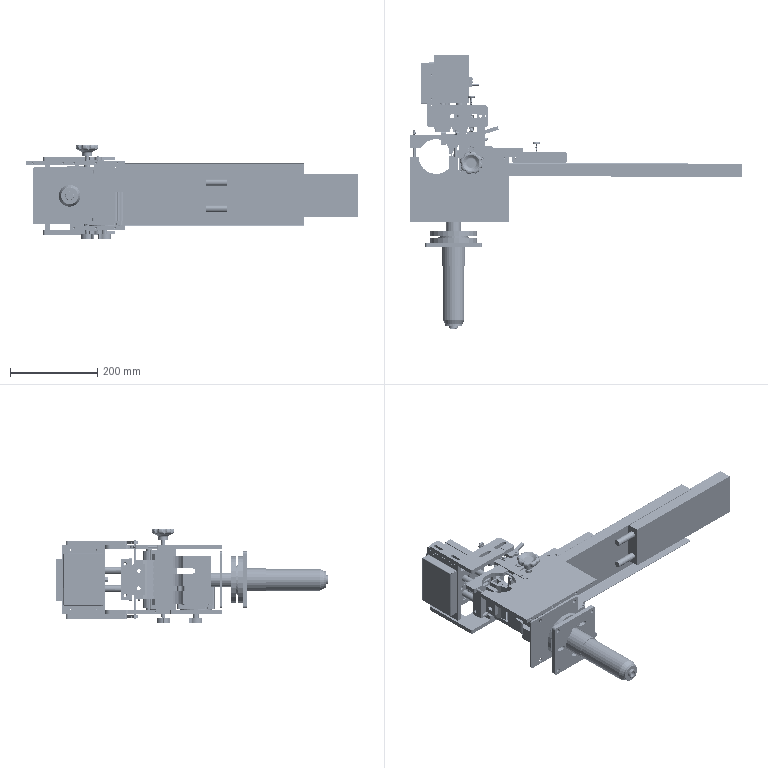Assembly | SolidWorks | mm | 70 component files | 73 solids | 4657 faces | box 762 x 626.5 x 217.5 mm | volume 5183306 mm3 | cylinder 2396 | plane 1290 | sphere 364 | torus 287 | cone 216 | spline 104 | commonest cylinder face diameters 4 x1072 6 x169 9 x90 0.4 x88 10 x69 5 x64 28 x58 30 x56
Bill of materials:
111.1 | 1 |  | Rectangular block-like plate with two holes drilled into one narrow edge face and two small holes through the broad face near one long side.
120.1 | 1 |  | Long slender bar with a thicker block at each end, giving a shallow C/bracket side profile, and four through holes spaced along its length.
121.1 | 1 |  | Thin flat plate whose ends are cut at angles, giving an irregular polygonal outline in one view, with two small through holes near one long edge.
86StepperMotor-XG2.1 | 1 |  | Square-section housing with a wider square flange at the base and a cylindrical shaft sticking out of the flange face; its overall form looks like a motor-style body.
113.1 | 1 |  | Rectangular block with a stepped profile (thick section narrowing through fillets to a thinner section) and two parallel obround through slots.
114.1 | 1 |  | Stepped cylindrical pin with a larger-diameter section, a thin radial collar, and a smaller-diameter section.
115.1 | 1 |  | Flat annular disc/flange with a large central bore and six holes on a circle, alternating between two sizes.
116.1 | 1 |  | Flat annular disc/flange with a large central bore, a step or recess around the bore on one face, and nine holes in three sizes on a circle.
117.1 | 1 |  | Thin flat ring (washer- or shim-like annulus) with a narrow radial width.
118.1 | 1 |  | Plain annular ring, thicker than a thin washer, with a narrow radial wall.
Ultrasonic.1 | 1 |  | Elongated cylindrical body with one end tapering through a conical chamfer to a smaller stepped boss and a small tubular nub with a central bore.
UltrasonicConnectionBlock.1 | 1 |  | Square flat plate with rounded corners, four corner through holes, a large central lobed opening, and three obround slots around the opening.
MainTailstock.1 | 2 |  | Flat, constant-thickness plate with a stepped, offset (Z-like) outline and rounded corners. It has five round through holes in the face and one small hole drilled into a side edge.
Part1.1 | 2 |  | Thick, roughly rectangular block. One end is cut as a concave arc, one corner has a large radius, and there is one round through hole.
ShortBoltM4.1 | 2 |  | Headed threaded fastener shape: a large, thin, disc-shaped head with rounded edges and a smooth (non-knurled) rim, on a coaxial straight shank that has external thread form along most of its length. Looks like a thumb screw or leveling-foot style screw.
ShortBoltM4.1 | 2 |  | Screw-like part: a short, wide disc-shaped head with rounded edges and a long, threaded-looking cylindrical shank. There are plain sections near the head and at the tip.
TailstockAdjustmentPlate.1 | 2 |  | Flat rectangular bar with three equally spaced round through holes in a line. One end is a concave arc and the other end has one large rounded corner.
TailstockAdjustmentSub-Plate.1 | 2 |  | Thick plate with one large rounded corner, a concave arc on the opposite end ending in a small hooked tip, and one round through hole.
TailstockAxisBar.1 | 4 |  | Plain, slender solid cylindrical rod with flat ends.
BladeHolderPlate.1 | 2 |  | Rectangular plate or block with rounded corners and two parallel obround (slotted) through holes.
CoverPlate.1_2 | 1 |  | Thin rectangular plate with rounded corners, four small round holes near the corners, and a large central obround or rounded-rectangle opening.
CoverPlate.1 | 1 |  | Formed thin-wall, sheet-like tray: a shallow rectangular recessed pan with walls, plus outward flanges at two opposite ends. Each flange has two obround slots.
Frame.1 | 2 |  | Flat L-shaped plate with rounded corners and four elongated slots, two along each leg.
FrameCutterBackingPlate.1 | 1 |  | Long, narrow, thin strip with a tab at each end. Each tab has a small round hole and an obround slot. A narrow formed lip or rib runs along one long edge.
FrameFrontMatchingPlate.1 | 1 |  | Plain rectangular bar or block with two round blind holes that appear to have conical drill-point bottoms.
FrameFrontPlate.1 | 1 |  | Thick rectangular plate with a central rectangular through cutout, a pattern of round through holes, and two holes drilled into one narrow edge.
FrameLeftPlate.1 | 1 |  | Flat plate with a stepped outline: a wide rectangular lower section and a narrower arm. It has a long rectangular slot, a large obround cutout, four elongated slots, and several round holes.
FramePlateSlider.1 | 2 |  | Rectangular block with rounded vertical corners, one large round through bore set toward one end, and four corner through holes.
FrameRightPlate.1 | 1 |  | Flat plate with a stepped outline: a wide solid rectangular section and a narrower arm with a long rectangular slot and several round holes. It has the same outline as unnamed part, but without the obround cutout and elongated slots.
GB_T276-94DeepGrooveBallBearing61800.1 | 4 | GCr4 | Ring-shaped assembly of concentric inner and outer rings with a ring of spherical balls between them; it looks like an open ball bearing.
Handle.1 | 2 |  | Straight bar of rectangular section with a semicircular lobe on one side; the lobe holds a round through hole. The lobe blends into the bar with fillets.
HeatingBlock.1 | 1 |  | Plain rectangular block with two parallel cylindrical pins sticking out of one end face.
HeatingBoxCover.1 | 1 |  | Long thin-walled channel (C-shaped section) made of a flat web and two short flanges, with small inner bend radii.
HotKnife.1 | 1 |  | Plate with a row of teeth along one long edge and two round through holes. In profile it tapers toward the toothed edge and has a rectangular notch on the opposite side; it looks like a serrated blade.
HotKnife-Copy.1 | 1 |  | Plate tapering to a single-bevel straight edge, with two round through holes and a rectangular notch in the thicker back portion of the profile; it looks like a straight-edged blade.
KnurledWheel.1 | 1 |  | Round knob with a scalloped (lobed) rim, a shallow dished top, and a conical underside that tapers into a cylindrical hub.
LongBoltM4.1 | 2 |  | Long, slender threaded rod with a flat cylindrical disc head at one end and a short neck between the head and the threads.
PatternedRoller.1 | 1 |  | Cylindrical roller-like body with stepped, smaller-diameter journals extending coaxially from both ends; faint helical lines on the main cylindrical surface.
PipeLockPlate.1 | 1 |  | Flat rectangular plate with a large circular opening at one end, split across the bore; a separate cap block closes the opening and is joined to the plate by two parallel rods with threaded ends, forming a split-bore clamp shape.
PryBarAxis.1 | 1 |  | Long, slender solid cylindrical rod with short modified sections at both ends.
Pulley11.1 | 1 |  | Short cylindrical toothed wheel with evenly spaced rectangular teeth around its outside and a central round through-bore that has one rectangular keyway. Looks like a simplified spur gear, sprocket or timing pulley with straight-sided teeth.
Pulley11.1 | 1 |  | Short cylindrical disk with evenly spaced rectangular teeth around its outside and a central round through-bore.
PunchingKnifeBackingPlate.1 | 2 |  | Flat rectangular plate with rounded corners, an elongated slot near each end, and two small round through-holes between the slots.
RubberRoller.1 | 1 |  | Plain cylindrical body with coaxial stepped journals at both ends.
Spring.1 | 2 |  | Helical coil of round wire with constant coil diameter and uniform pitch, ends left open.
CS1-J().1 | 2 |  | Multi-feature body: a rectangular base block with a raised open-frame upright holding a short cross pin, a long cylindrical rod sticking out sideways, rounded bosses on one face, and a thin hooked lip.
TN32-30 - 30_b.1 | 2 |  | Rectangular block with two parallel stacked bores on one end face, longitudinal grooves on several faces, through-holes on the broad face, and a protruding hex-shaped fitting.
TN32-30_fp.1 | 2 |  | Rectangular end plate carrying two parallel cylindrical rods, each ending in a larger-diameter cylindrical head.
Mates:
1. symmetric | FrameLeftPlate.1-1 face at (2, 116, -70) dir (0, 0, 1) | FrameRightPlate.1-1 face at (2, 116, 70) dir (0, 0, -1) | assembly plane at (0, 0, 0) dir (0, 0, 1)
2. concentric | FrameLeftPlate.1-1 face at (67, 146, -70) dir (0, 0, 1) r 2.75 | 111.1-1 face at (67, 146, -70) dir (0, 0, -1) r 2.1
3. width | 111.1-1 face at (127, 150, -70) dir (0, 0, -1) | 111.1-1 face at (127, 150, 70) dir (0, 0, 1) | FrameLeftPlate.1-1 face at (2, 116, -70) dir (0, 0, 1) | FrameRightPlate.1-1 face at (2, 116, 70) dir (0, 0, -1)
4. concentric | FrameRightPlate.1-1 face at (17, 116.5, 79.4) dir (0, 0, 1) r 2.75 | FrameFrontMatchingPlate.1-1 face at (17, 116.5, 70) dir (0, 0, 1) r 2.1
5. concentric | FrameLeftPlate.1-1 face at (17, 131.5, -70) dir (0, 0, 1) r 2.75 | FrameFrontMatchingPlate.1-1 face at (17, 131.5, -70) dir (0, 0, -1) r 2.1
6. width | FrameFrontMatchingPlate.1-1 face at (21, 146.5, -70) dir (0, 0, -1) | FrameFrontMatchingPlate.1-1 face at (21, 146.5, 70) dir (0, 0, 1) | FrameLeftPlate.1-1 face at (2, 116, -70) dir (0, 0, 1) | FrameRightPlate.1-1 face at (2, 116, 70) dir (0, 0, -1)
7. coincident | FrameLeftPlate.1-1 face at (10, 268, -70) dir (0, 1, 0) | Frame.1-1 face at (69.5, 268, -79.4) dir (0, 1, 0)
8. coincident | FrameLeftPlate.1-1 face at (2, 116, -79.4) dir (0, 0, -1) | Frame.1-1 face at (69.5, 258, -79.4) dir (0, 0, 1)
9. coincident | FrameRightPlate.1-1 face at (10, 268, 79.4) dir (0, 1, 0) | Frame.1-2 face at (69.5, 268, 89.4) dir (0, 1, 0)
10. coincident | FrameRightPlate.1-1 face at (2, 116, 79.4) dir (0, 0, 1) | Frame.1-2 face at (69.5, 258, 79.4) dir (0, 0, -1)
11. width | FrameFrontPlate.1-1 face at (-55.5, 363, -79.4) dir (0, 0, -1) | FrameFrontPlate.1-1 face at (-55.5, 363, 79.4) dir (0, 0, 1) | Frame.1-1 face at (69.5, 258, -79.4) dir (0, 0, 1) | Frame.1-2 face at (69.5, 258, 79.4) dir (0, 0, -1)
12. coincident | FrameFrontMatchingPlate.1-1 face at (21, 146.5, 70) dir (0, 1, 0) | FrameCutterBackingPlate.1-1 face at (0, 146.5, -69) dir (0, -1, 0)
13. width | FrameCutterBackingPlate.1-1 face at (34, 150.5, 69) dir (0, 0, 1) | FrameCutterBackingPlate.1-1 face at (34, 150.5, -69) dir (0, 0, -1) | FrameRightPlate.1-1 face at (2, 116, 70) dir (0, 0, -1) | FrameLeftPlate.1-1 face at (2, 116, -70) dir (0, 0, 1)
14. coincident | 120.1-1 face at (2, 150.5, 69) dir (0, -1, 0) | FrameCutterBackingPlate.1-1 face at (0, 150.5, -69) dir (0, 1, 0)
15. concentric | 120.1-1 face at (8, 150.5, -63) dir (0, -1, 0) r 2.5 | FrameCutterBackingPlate.1-1 face at (8, 146.5, -63) dir (0, -1, 0) r 1.65
16. coincident | 120.1-1 face at (0, 159.5, 59) dir (0, -1, 0) | 121.1-1 face at (5, 159.5, -58) dir (0, 1, 0)
17. concentric | FrameRightPlate.1-1 face at (40.5, 135, 79.4) dir (0, 0, -1) r 9.5 | PatternedRoller.1-1 face at (40.5, 135, 70) dir (0, 0, -1) r 7
18. width | PatternedRoller.1-1 face at (40.5, 135, -65) dir (0, 0, -1) | PatternedRoller.1-1 face at (40.5, 135, 65) dir (0, 0, 1) | FrameRightPlate.1-1 face at (2, 116, 79.4) dir (0, 0, 1) | FrameLeftPlate.1-1 face at (2, 116, -79.4) dir (0, 0, -1)
19. concentric | FrameRightPlate.1-1 face at (40.5, 268, 74.7) dir (0, 1, 0) r 2.1 | LongBoltM4.1-1 face at (40.5, 290, 74.7) dir (0, -1, 0) r 8
20. distance | FrameRightPlate.1-1 face at (10, 268, 79.4) dir (0, 1, 0) | LongBoltM4.1-1 face at (40.5, 290, 74.7) dir (0, 1, 0)
21. coincident | Spring.1-1 plane at (40.5, 207.5, 74.7) dir (0.3882, 0, 0.9216) | LongBoltM4.1-1 plane at (40.5, 205, 74.7) dir (0.3882, 0, 0.9216)
22. coincident | Spring.1-1 plane at (40.5, 207.5, 74.7) dir (0.9216, 0, -0.3882) | LongBoltM4.1-1 plane at (40.5, 205, 74.7) dir (-0.9216, 0, 0.3882)
23. concentric | FrameLeftPlate.1-1 face at (40.5, 268, -74.7) dir (0, 1, 0) r 2.1 | LongBoltM4.1-2 face at (40.5, 290, -74.7) dir (0, -1, 0) r 8
24. distance | LongBoltM4.1-2 face at (40.5, 290, -74.7) dir (0, 1, 0) | FrameLeftPlate.1-1 face at (10, 268, -70) dir (0, 1, 0)
25. coincident | LongBoltM4.1-2 plane at (40.5, 205, -74.7) dir (0.3882, 0, 0.9216) | Spring.1-2 plane at (40.5, 207.5, -74.7) dir (0.3882, 0, 0.9216)
26. coincident | LongBoltM4.1-2 plane at (40.5, 205, -74.7) dir (-0.9216, 0, 0.3882) | Spring.1-2 plane at (40.5, 207.5, -74.7) dir (0.9216, 0, -0.3882)
27. width | FramePlateSlider.1-1 face at (27.5, 205.5, 70) dir (-1, 0, 0) | FramePlateSlider.1-1 face at (53.5, 205.5, 70) dir (1, 0, 0) | FrameRightPlate.1-1 face at (53.5, 248, 79.4) dir (-1, 0, 0) | FrameRightPlate.1-1 face at (27.5, 248, 79.4) dir (1, 0, 0)
28. distance | FrameRightPlate.1-1 face at (29.5, 148, 79.4) dir (0, 1, 0) | FramePlateSlider.1-1 face at (51.5, 151.5, 70) dir (0, -1, 0)
29. coincident | FrameRightPlate.1-1 face at (2, 116, 79.4) dir (0, 0, 1) | FramePlateSlider.1-1 face at (29.5, 153.5, 79.4) dir (0, 0, 1)
30. width | FramePlateSlider.1-2 face at (53.5, 205.5, -70) dir (1, 0, 0) | FramePlateSlider.1-2 face at (27.5, 205.5, -70) dir (-1, 0, 0) | FrameLeftPlate.1-1 face at (27.5, 248, -70) dir (1, 0, 0) | FrameLeftPlate.1-1 face at (53.5, 248, -70) dir (-1, 0, 0)
31. coincident | FrameLeftPlate.1-1 face at (2, 116, -79.4) dir (0, 0, -1) | FramePlateSlider.1-2 face at (51.5, 153.5, -79.4) dir (0, 0, -1)
32. concentric | FrameLeftPlate.1-1 face at (40.5, 135, -70) dir (0, 0, -1) r 9.5 | GB_T276-94DeepGrooveBallBearing61800.1-3 face at (40.5, 135, -72.5) dir (0, 0, 1) r 9.5
33. concentric | FrameRightPlate.1-1 face at (40.5, 135, 79.4) dir (0, 0, -1) r 9.5 | GB_T276-94DeepGrooveBallBearing61800.1-2 face at (40.5, 135, 72.5) dir (0, 0, 1) r 9.5
34. concentric | KnurledWheel.1-1 face at (40.5, 135, 92) dir (0, 0, -1) r 4 | PatternedRoller.1-1 face at (40.5, 135, 100) dir (0, 0, -1) r 4
35. coincident | FramePlateSlider.1-1 face at (51.5, 207.5, 70) dir (0, 1, 0) | Spring.1-1 plane at (40.5, 207.5, 74.7) dir (0, -1, 0)
36. coincident | FramePlateSlider.1-2 face at (29.5, 207.5, -70) dir (0, 1, 0) | Spring.1-2 plane at (40.5, 207.5, -74.7) dir (0, -1, 0)
37. concentric | FrameRightPlate.1-1 face at (65, 200, 79.4) dir (0, 0, -1) r 3 | PryBarAxis.1-1 face at (65, 200, 90) dir (0, 0, -1) r 3
38. width | FrameRightPlate.1-1 face at (2, 116, 79.4) dir (0, 0, 1) | FrameLeftPlate.1-1 face at (2, 116, -79.4) dir (0, 0, -1) | PryBarAxis.1-1 face at (65, 200, -90) dir (0, 0, -1) | PryBarAxis.1-1 face at (65, 200, 90) dir (0, 0, 1)
39. width | FrameFrontPlate.1-1 face at (-55.5, 363, -74.4) dir (-1, 0, 0) | FrameFrontPlate.1-1 face at (-45.5, 363, -74.4) dir (1, 0, 0) | Frame.1-1 face at (-54, 346, -79.4) dir (1, 0, 0) | Frame.1-1 face at (-47, 346, -79.4) dir (-1, 0, 0)
40. concentric | PunchingKnifeBackingPlate.1-1 face at (-22.75, 214, -27.5) dir (0, 1, 0) r 2.75 | BladeHolderPlate.1-2 face at (-22.75, 206, -27.5) dir (0, 1, 0) r 2.1
41. concentric | PunchingKnifeBackingPlate.1-1 face at (-22.75, 214, 27.5) dir (0, 1, 0) r 2.75 | BladeHolderPlate.1-2 face at (-22.75, 206, 27.5) dir (0, 1, 0) r 2.1
42. coincident | PunchingKnifeBackingPlate.1-1 face at (-10.75, 206, 47) dir (0, -1, 0) | BladeHolderPlate.1-2 face at (-27.75, 206, -33) dir (0, 1, 0)
43. coincident | HotKnife.1-1 face at (-17.75, 201, -45) dir (-1, 0, 0) | BladeHolderPlate.1-2 face at (-17.75, 178, -33) dir (1, 0, 0)
44. coincident | HotKnife-Copy.1-1 face at (6.75, 201, 45) dir (1, 0, 0) | BladeHolderPlate.1-3 face at (6.75, 178, 33) dir (-1, 0, 0)
45. coincident | Frame.1-1 face at (-60.5, 353, -79.4) dir (-1, 0, 0) | Frame.1-2 face at (-60.5, 353, 89.4) dir (-1, 0, 0)
46. concentric | 120.1-1 face at (8, 150.5, 63) dir (0, -1, 0) r 2.5 | FrameCutterBackingPlate.1-1 face at (8, 146.5, 63) dir (0, -1, 0) r 1.65
47. concentric | 120.1-1 face at (8, 164.5, 40) dir (0, 1, 0) r 2.5 | 121.1-1 face at (8, 159.5, 40) dir (0, 1, 0) r 1.65
48. concentric | 120.1-1 face at (8, 164.5, -40) dir (0, 1, 0) r 2.5 | 121.1-1 face at (8, 159.5, -40) dir (0, 1, 0) r 1.65
49. distance | FrameCutterBackingPlate.1-1 face at (12, 150.5, -57.5) dir (-1, 0, 0) | FrameFrontMatchingPlate.1-1 face at (13, 106.5, -70) dir (-1, 0, 0)
50. width | RubberRoller.1-1 face at (40.5, 166.5, 65) dir (0, 0, 1) | RubberRoller.1-1 face at (40.5, 166.5, -65) dir (0, 0, -1) | FramePlateSlider.1-1 face at (29.5, 153.5, 70) dir (0, 0, -1) | FramePlateSlider.1-2 face at (51.5, 153.5, -70) dir (0, 0, 1)
51. distance | FrameRightPlate.1-1 face at (2, 116, 79.4) dir (0, 0, 1) | FrameLeftPlate.1-1 face at (2, 116, -79.4) dir (0, 0, -1)
52. distance | HotKnife-Copy.1-1 face at (-5.25, 201, 45) dir (0, 1, 0) | BladeHolderPlate.1-3 face at (16.75, 176, 33) dir (0, -1, 0)
53. distance | BladeHolderPlate.1-2 face at (-27.75, 176, -33) dir (0, -1, 0) | HotKnife.1-1 face at (-5.75, 201, -45) dir (0, 1, 0)
54. width | HotKnife-Copy.1-1 face at (6.75, 201, -45) dir (0, 0, -1) | HotKnife-Copy.1-1 face at (6.75, 201, 45) dir (0, 0, 1) | BladeHolderPlate.1-3 face at (16.75, 204, 35) dir (0, 0, 1) | BladeHolderPlate.1-3 face at (16.75, 204, -35) dir (0, 0, -1)
55. concentric | PryBarAxis.1-1 face at (65, 200, 90) dir (0, 0, -1) r 3 | Handle.1-1 face at (65, 200, -82) dir (0, 0, -1) r 3
56. distance | PryBarAxis.1-1 face at (65, 200, 90) dir (0, 0, 1) | Handle.1-2 face at (55.803, 193.966, 88) dir (0, 0, 1)
57. distance | PryBarAxis.1-1 face at (65, 200, -90) dir (0, 0, -1) | Handle.1-1 face at (55.797, 193.975, -88) dir (0, 0, -1)
58. concentric | FrameFrontPlate.1-1 face at (-55.5, 356, 0) dir (-1, 0, 0) r 2.5 | TN32X30S(0)+(CS1-J-1).1-1/TN32-30 - 30_b.1-1 face at (-45.5, 356, 0) dir (1, 0, 0) r 4.5
59. concentric | FrameFrontPlate.1-1 face at (-55.5, 291, 0) dir (-1, 0, 0) r 2.5 | TN32X30S(0)+(CS1-J-1).1-1/TN32-30 - 30_b.1-1 face at (-45.5, 291, 0) dir (1, 0, 0) r 2.75
60. coincident | FrameFrontPlate.1-1 face at (-45.5, 363, -74.4) dir (1, 0, 0) | TN32X30S(0)+(CS1-J-1).1-1/TN32-30 - 30_b.1-1 face at (-45.5, 382, 3.95) dir (-1, 0, 0)
61. concentric | FrameFrontPlate.1-1 face at (-55.5, 329, -41.5) dir (-1, 0, 0) r 2.5 | TN32X30S(0)+(CS1-J-1).1-2/TN32-30 - 30_b.1-1 edge at (-5.5, 329, -41.5) dir (-1, 0, 0) r 4.5
62. concentric | FrameFrontPlate.1-1 face at (-55.5, 356, 0) dir (-1, 0, 0) r 2.5 | TN32X30S(0)+(CS1-J-1).1-2/TN32-30 - 30_b.1-1 face at (-5.5, 356, 0) dir (1, 0, 0) r 4.5
63. coincident | TN32X30S(0)+(CS1-J-1).1-1/TN32-30 - 30_b.1-1 face at (-5.5, 382, 48) dir (1, 0, 0) | TN32X30S(0)+(CS1-J-1).1-2/TN32-30 - 30_b.1-1 face at (-5.5, 382, 3.95) dir (-1, 0, 0)
64. coincident | PunchingKnifeBackingPlate.1-1 face at (-10.75, 214, 47) dir (0, 1, 0) | TN32X30S(0)+(CS1-J-1).1-1/TN32-30_fp.1-1 face at (-44.5, 214, 0) dir (0, -1, 0)
65. width | PunchingKnifeBackingPlate.1-3 face at (-0.25, 214, 49) dir (0, 0, 1) | PunchingKnifeBackingPlate.1-3 face at (-0.25, 214, -49) dir (0, 0, -1) | TN32X30S(0)+(CS1-J-1).1-2/TN32-30_fp.1-1 face at (33.3, 231, -47) dir (0, 0, -1) | TN32X30S(0)+(CS1-J-1).1-2/TN32-30_fp.1-1 face at (-4.3, 231, 47) dir (0, 0, 1)
66. coincident | TN32X30S(0)+(CS1-J-1).1-2/TN32-30_fp.1-1 face at (-4.5, 214, 0) dir (0, -1, 0) | PunchingKnifeBackingPlate.1-3 face at (-0.25, 214, -47) dir (0, 1, 0)
67. concentric | BladeHolderPlate.1-3 face at (11.75, 206, -27.5) dir (0, 1, 0) r 2.1 | PunchingKnifeBackingPlate.1-3 face at (11.75, 214, -27.5) dir (0, 1, 0) r 2.75
68. concentric | BladeHolderPlate.1-3 edge at (11.75, 206, 27.5) dir (0, 1, 0) r 2.1 | PunchingKnifeBackingPlate.1-3 face at (11.75, 214, 27.5) dir (0, 1, 0) r 2.75
69. distance | PunchingKnifeBackingPlate.1-1 face at (-42.75, 214, -47) dir (-1, 0, 0) | TN32X30S(0)+(CS1-J-1).1-1/TN32-30_fp.1-1 face at (-44.5, 231, -46.8) dir (-1, 0, 0)
70. distance | TN32X30S(0)+(CS1-J-1).1-2/TN32-30_fp.1-1 face at (33.5, 231, 46.8) dir (1, 0, 0) | PunchingKnifeBackingPlate.1-3 face at (31.75, 214, 47) dir (1, 0, 0)
71. concentric | BladeHolderPlate.1-3 face at (11.75, 206, 27.5) dir (0, 1, 0) r 2.1 | PunchingKnifeBackingPlate.1-3 face at (11.75, 214, 27.5) dir (0, 1, 0) r 2.75
72. concentric | BladeHolderPlate.1-3 face at (11.75, 206, -27.5) dir (0, 1, 0) r 2.1 | PunchingKnifeBackingPlate.1-3 face at (11.75, 214, -27.5) dir (0, 1, 0) r 2.75
73. coincident | BladeHolderPlate.1-3 face at (16.75, 206, 33) dir (0, 1, 0) | PunchingKnifeBackingPlate.1-3 face at (-0.25, 206, -47) dir (0, -1, 0)
74. distance | Frame.1-1 face at (-35.5, 358, -79.4) dir (0, 1, 0) | FrameFrontPlate.1-1 face at (-55.5, 368, -74.4) dir (0, 1, 0)
75. distance | Frame.1-2 face at (79.5, 223, 89.4) dir (1, 0, 0) | FrameRightPlate.1-1 face at (72, 258, 79.4) dir (1, 0, 0)
76. concentric | PryBarAxis.1-1 face at (65, 200, 90) dir (0, 0, -1) r 3 | Handle.1-2 face at (65, 200, 88) dir (0, 0, -1) r 3
77. concentric | PatternedRoller.1-1 face at (40.5, 135, 100) dir (0, 0, -1) r 4 | Pulley11.1-2 face at (40.5, 135, -88) dir (0, 0, -1) r 4
78. coincident | PatternedRoller.1-1 face at (40.5, 135, -100) dir (0, 0, -1) | Pulley11.1-2 face at (40.5, 135, -100) dir (0, 0, -1)
79. concentric | FramePlateSlider.1-1 face at (40.5, 166.5, 70) dir (0, 0, 1) r 7.5 | RubberRoller.1-1 face at (40.5, 166.5, -80) dir (0, 0, 1) r 5
80. concentric | FramePlateSlider.1-2 face at (40.5, 166.5, -70) dir (0, 0, -1) r 7.5 | RubberRoller.1-1 face at (40.5, 166.5, -80) dir (0, 0, 1) r 5
81. coincident | FrameLeftPlate.1-1 face at (0, 0, -70) dir (0, -1, 0) | assembly plane at (0, 0, 0) dir (0, 1, 0)
82. distance | 86StepperMotor-XG2.1-1 plane at (80.5, 60, -58.5) dir (1, 0, 0) | FrameLeftPlate.1-1 face at (127, 0, -70) dir (1, 0, 0)
83. coincident | FrameLeftPlate.1-1 face at (0, 0, -70) dir (-1, 0, 0) | assembly plane at (0, 0, 0) dir (1, 0, 0)
84. distance | 86StepperMotor-XG2.1-1 plane at (80.5, 60, -58.5) dir (0, 1, 0) | FrameLeftPlate.1-1 face at (0, 0, -70) dir (0, -1, 0)
85. coincident | FrameLeftPlate.1-1 face at (2, 116, -70) dir (0, 0, 1) | 86StepperMotor-XG2.1-1 face at (80.5, 60, -70) dir (0, 0, -1)
86. coincident | PatternedRoller.1-1 face at (40.5, 135, 70) dir (0, 0, 1) | GB_T276-94DeepGrooveBallBearing61800.1-2 face at (42.679, 140.911, 70) dir (0, 0, -1)
87. coincident | PatternedRoller.1-1 face at (40.5, 135, -70) dir (0, 0, -1) | GB_T276-94DeepGrooveBallBearing61800.1-3 face at (40.5, 141.3, -70) dir (0, 0, 1)
88. concentric | FramePlateSlider.1-1 face at (40.5, 166.5, 75) dir (0, 0, -1) r 9.5 | GB_T276-94DeepGrooveBallBearing61800.1-4 face at (40.5, 166.5, 72.5) dir (0, 0, 1) r 9.5
89. coincident | FramePlateSlider.1-1 face at (40.5, 166.5, 75) dir (0, 0, -1) | GB_T276-94DeepGrooveBallBearing61800.1-4 face at (43.682, 175.132, 75) dir (0, 0, 1)
90. concentric | FramePlateSlider.1-2 face at (40.5, 166.5, -75) dir (0, 0, 1) r 9.5 | GB_T276-94DeepGrooveBallBearing61800.1-5 face at (40.5, 166.5, -72.5) dir (0, 0, 1) r 9.5
91. coincident | FramePlateSlider.1-2 face at (40.5, 166.5, -75) dir (0, 0, 1) | GB_T276-94DeepGrooveBallBearing61800.1-5 face at (40.502, 175.7, -75) dir (0, 0, -1)
92. concentric | Assembly5.1-1/MainTailstock.1-1 face at (105, 170, -64.5) dir (0, 1, 0) r 2.1 | 111.1-1 face at (105, 150, -64.5) dir (0, 1, 0) r 1.65
93. parallel | Assembly5.1-1/MainTailstock.1-1 face at (255, 140, -61.5) dir (0, 0, 1) | FrameLeftPlate.1-1 face at (2, 116, -70) dir (0, 0, 1)
94. coincident | Assembly5.1-1/MainTailstock.1-1 face at (130, 150, -61.5) dir (0, -1, 0) | 111.1-1 face at (57, 150, 70) dir (0, 1, 0)
95. coincident | FrameFrontPlate.1-1 face at (-55.5, 363, -74.4) dir (-1, 0, 0) | CoverPlate.1-1 face at (-55.5, 318, 0) dir (1, 0, 0)
96. width | CoverPlate.1-1 face at (-75.5, 364, 0) dir (0, 1, 0) | CoverPlate.1-1 face at (-75.5, 272, 0) dir (0, -1, 0) | FrameFrontPlate.1-1 face at (-55.5, 268, -79.4) dir (0, -1, 0) | FrameFrontPlate.1-1 face at (-55.5, 368, -74.4) dir (0, 1, 0)
97. width | CoverPlate.1-1 face at (-75.5, 318, 60) dir (0, 0, 1) | CoverPlate.1-1 face at (-75.5, 318, -60) dir (0, 0, -1) | Frame.1-1 face at (69.5, 258, -89.4) dir (0, 0, -1) | Frame.1-2 face at (69.5, 258, 89.4) dir (0, 0, 1)
98. coincident | FrameRightPlate.1-1 face at (0, 0, 79.4) dir (-1, 0, 0) | PipeLockPlate.1-1 face at (0, 118, 79.4) dir (1, 0, 0)
99. coincident | FrameRightPlate.1-1 face at (2, 116, 79.4) dir (0, 0, 1) | PipeLockPlate.1-1 face at (-40, 150, 79.4) dir (0, 0, 1)
100. coincident | Assembly5.1-1/MainTailstock.1-2 face at (255, 135, 67.5) dir (0, -1, 0) | HeatingBoxCover.1-1 face at (127, 135, 75.621) dir (0, 1, 0)
101. coincident | FrameRightPlate.1-1 face at (127, 0, 79.4) dir (1, 0, 0) | HeatingBoxCover.1-1 face at (127, 132.5, -68.879) dir (-1, 0, 0)
102. coincident | HeatingBoxCover.1-1 face at (127, 133.5, 75.621) dir (0, -1, 0) | HeatingBlock.1-1 face at (362, 133.5, -50) dir (0, 1, 0)
103. concentric | FramePlateSlider.1-2 face at (40.5, 166.5, -70) dir (0, 0, -1) r 7.5 | RubberRoller.1-1 face at (40.5, 166.5, 70) dir (0, 0, -1) r 15.5
104. concentric | 86StepperMotor-XG2.1-1 face at (80.5, 60, -100.5) dir (0, 0, 1) r 6.35 | Pulley11.1-1 face at (80.5, 60, -79.5) dir (0, 0, -1) r 6.4
105. concentric | 114.1-1 face at (-33.045, -47.107, 0) dir (0, -1, 0) r 16.5 | 115.1-1 face at (-33.045, -110.107, 0) dir (0, -1, 0) r 29
106. concentric | 114.1-1 face at (-33.045, -47.107, 0) dir (0, -1, 0) r 16.5 | 116.1-1 face at (-33.045, -104.107, 0) dir (0, 1, 0) r 29
107. concentric | 114.1-1 face at (-33.045, -47.107, 0) dir (0, -1, 0) r 16.5 | 118.1-1 face at (-33.045, -106.107, 0) dir (0, -1, 0) r 35
108. concentric | 114.1-1 face at (-33.045, -47.107, 0) dir (0, -1, 0) r 16.5 | 117.1-1 face at (-33.045, -104.107, 0) dir (0, 1, 0) r 35
109. coincident | 113.1-1 face at (-88.045, -47.107, 22) dir (0, -1, 0) | 114.1-1 face at (-33.045, -47.107, 0) dir (0, 1, 0)
110. symmetric | 113.1-1 face at (21.955, -47.107, -22) dir (0, 0, -1) | 113.1-1 face at (21.955, -47.107, 22) dir (0, 0, 1) | 114.1-1 plane at (-33.045, -104.107, 0) dir (0, 0, 1)
111. symmetric | 113.1-1 face at (-88.045, 77.893, 22) dir (-1, 0, 0) | 113.1-1 face at (21.955, 77.893, 22) dir (1, 0, 0) | 114.1-1 plane at (-33.045, -104.107, 0) dir (1, 0, 0)
112. coincident | 114.1-1 face at (-33.045, -174.107, 0) dir (0, -1, 0) | Ultrasonic.1-1 face at (-33.045, -174.107, 0) dir (0, 1, 0)
113. concentric | 114.1-1 face at (-33.045, -174.107, 0) dir (0, 1, 0) r 27 | Ultrasonic.1-1 face at (-33.045, -82.454, 0) dir (0, 1, 0) r 25
114. coincident | 114.1-1 face at (-33.045, -104.107, 0) dir (0, 1, 0) | 117.1-1 face at (-33.045, -104.107, 0) dir (0, -1, 0)
115. coincident | 114.1-1 face at (-33.045, -108.107, 0) dir (0, -1, 0) | 118.1-1 face at (-33.045, -108.107, 0) dir (0, 1, 0)
116. coincident | 115.1-1 face at (-33.045, -112.107, 0) dir (0, 1, 0) | 118.1-1 face at (-33.045, -112.107, 0) dir (0, -1, 0)
117. coincident | 116.1-1 face at (-33.045, -102.107, 0) dir (0, -1, 0) | 117.1-1 face at (-33.045, -102.107, 0) dir (0, 1, 0)
118. concentric | Ultrasonic.1-1 face at (-33.045, -82.454, 0) dir (0, 1, 0) r 25 | UltrasonicConnectionBlock.1-1 face at (-33.045, -120.107, 0) dir (0, -1, 0) r 30
119. coincident | 114.1-1 plane at (-33.045, -104.107, 0) dir (1, 0, 0) | 115.1-1 plane at (-33.045, -120.107, 0) dir (-1, 0, 0)
120. coincident | 114.1-1 plane at (-33.045, -104.107, 0) dir (1, 0, 0) | UltrasonicConnectionBlock.1-1 plane at (-33.045, -130.107, 0) dir (1, 0, 0)
121. coincident | 115.1-1 face at (-33.045, -120.107, 0) dir (0, -1, 0) | UltrasonicConnectionBlock.1-1 face at (26.955, -120.107, -60) dir (0, 1, 0)
122. symmetric | MainTailstock.1-1 face at (-5, 5, -61.5) dir (0, 0, 1) | MainTailstock.1-2 face at (-5, 5, 61.5) dir (0, 0, -1) | Assembly5.1 plane at (0, 0, 0) dir (0, 0, 1)
123. distance | MainTailstock.1-2 face at (-5, 5, 67.5) dir (0, 0, 1) | MainTailstock.1-1 face at (-5, 5, -67.5) dir (0, 0, -1)
124. coincident | MainTailstock.1-1 face at (-98, 25, -61.5) dir (0, 1, 0) | MainTailstock.1-2 face at (-98, 25, 67.5) dir (0, 1, 0)
125. concentric | MainTailstock.1-1 face at (-190, 29, -61.5) dir (0, 0, -1) r 3 | MainTailstock.1-2 face at (-190, 29, 67.5) dir (0, 0, -1) r 3
126. concentric | MainTailstock.1-1 face at (-10, 10, -61.5) dir (0, 0, -1) r 3 | MainTailstock.1-2 face at (-10, 10, 67.5) dir (0, 0, -1) r 3
127. concentric | MainTailstock.1-2 face at (-190, 29, 67.5) dir (0, 0, -1) r 3 | TailstockAxisBar.1-1 face at (-190, 29, 67.5) dir (0, 0, -1) r 3
128. concentric | MainTailstock.1-1 face at (-70, 10, -61.5) dir (0, 0, -1) r 3 | TailstockAxisBar.1-3 face at (-70, 10, 67.5) dir (0, 0, -1) r 3
129. concentric | MainTailstock.1-1 face at (-40, 10, -61.5) dir (0, 0, -1) r 3 | TailstockAxisBar.1-4 face at (-40, 10, 67.5) dir (0, 0, -1) r 3
130. concentric | MainTailstock.1-1 face at (-10, 10, -61.5) dir (0, 0, -1) r 3 | TailstockAxisBar.1-5 face at (-10, 10, 67.5) dir (0, 0, -1) r 3
131. coincident | MainTailstock.1-1 face at (-5, 5, -67.5) dir (0, 0, -1) | TailstockAxisBar.1-5 face at (-10, 10, -67.5) dir (0, 0, -1)
132. coincident | MainTailstock.1-1 face at (-5, 5, -67.5) dir (0, 0, -1) | TailstockAxisBar.1-4 face at (-40, 10, -67.5) dir (0, 0, -1)
133. coincident | MainTailstock.1-1 face at (-5, 5, -67.5) dir (0, 0, -1) | TailstockAxisBar.1-3 face at (-70, 10, -67.5) dir (0, 0, -1)
134. coincident | MainTailstock.1-1 face at (-5, 5, -67.5) dir (0, 0, -1) | TailstockAxisBar.1-1 face at (-190, 29, -67.5) dir (0, 0, -1)
135. concentric | TailstockAxisBar.1-3 face at (-70, 10, 67.5) dir (0, 0, -1) r 3 | TailstockAdjustmentPlate.1-1 face at (-70, 10, 13.563) dir (0, 0, -1) r 3.25
136. concentric | TailstockAxisBar.1-3 face at (-70, 10, 67.5) dir (0, 0, -1) r 3 | TailstockAdjustmentPlate.1-2 face at (-70, 10, -14.366) dir (0, 0, -1) r 3.25
137. concentric | TailstockAxisBar.1-4 face at (-40, 10, 67.5) dir (0, 0, -1) r 3 | TailstockAdjustmentPlate.1-1 edge at (-40, 10, 13.563) dir (0, 0, 1) r 3.25
138. concentric | TailstockAxisBar.1-4 face at (-40, 10, 67.5) dir (0, 0, -1) r 3 | TailstockAdjustmentPlate.1-2 edge at (-40, 10, -14.366) dir (0, 0, 1) r 3.25
139. concentric | TailstockAxisBar.1-1 face at (-190, 29, 67.5) dir (0, 0, -1) r 3 | TailstockAdjustmentSub-Plate.1-1 face at (-190, 29, -39.124) dir (0, 0, -1) r 3.25
140. concentric | TailstockAxisBar.1-1 face at (-190, 29, 67.5) dir (0, 0, -1) r 3 | TailstockAdjustmentSub-Plate.1-2 face at (-190, 29, 9.508) dir (0, 0, -1) r 3.25
141. concentric | TailstockAdjustmentSub-Plate.1-2 face at (-189.972, 36.5, 6.508) dir (0.003779, 1, 0) r 2 | ShortBoltM4.1-1 face at (-189.894, 57.05, 6.508) dir (-0.003779, -1, 0) r 8
142. distance | ShortBoltM4.1-1 face at (-189.894, 57.05, 6.508) dir (0.003779, 1, 0) | TailstockAdjustmentSub-Plate.1-2 face at (-177.972, 36.455, 9.508) dir (0.003779, 1, 0)
143. concentric | TailstockAdjustmentPlate.1-2 face at (-70, 18.5, -17.366) dir (0, 1, 0) r 2 | ShortBoltM4.1-3 face at (-70, 48.05, -17.366) dir (0, -1, 0) r 8
144. distance | ShortBoltM4.1-3 face at (-70, 48.05, -17.366) dir (0, 1, 0) | TailstockAdjustmentPlate.1-2 face at (-32, 18.5, -14.366) dir (0, 1, 0)
145. concentric | TailstockAdjustmentPlate.1-1 face at (-70, 18.5, 10.563) dir (0, 1, 0) r 2 | ShortBoltM4.1-4 face at (-70, 48.05, 10.563) dir (0, -1, 0) r 8
146. distance | ShortBoltM4.1-4 face at (-70, 48.05, 10.563) dir (0, 1, 0) | TailstockAdjustmentPlate.1-1 face at (-32, 18.5, 13.563) dir (0, 1, 0)
147. concentric | TailstockAdjustmentSub-Plate.1-1 face at (-190, 36.5, -42.124) dir (0, 1, 0) r 2 | ShortBoltM4.1-2 face at (-190, 57.05, -42.124) dir (0, -1, 0) r 8
148. distance | ShortBoltM4.1-2 face at (-190, 57.05, -42.124) dir (0, 1, 0) | TailstockAdjustmentSub-Plate.1-1 face at (-178, 36.5, -39.124) dir (0, 1, 0)
149. concentric | TailstockAxisBar.1-1 face at (-190, 29, 67.5) dir (0, 0, -1) r 3 | Part1.1-1 face at (-190, 29, 19.741) dir (0, 0, -1) r 3
150. parallel | MainTailstock.1-2 face at (-130, 15, 67.5) dir (0, -1, 0) | Part1.1-1 face at (-209.4, 15, 19.741) dir (0, -1, 0)
151. coincident | MainTailstock.1-1 face at (0, 20, -61.5) dir (1, 0, 0) | Assembly5.1 plane at (0, 0, 0) dir (1, 0, 0)
152. coincident | MainTailstock.1-2 face at (-5, 0, 67.5) dir (0, -1, 0) | Assembly5.1 plane at (0, 0, 0) dir (0, 1, 0)
153. concentric | TailstockAxisBar.1-1 face at (-190, 29, 67.5) dir (0, 0, -1) r 3 | Part1.1-2 face at (-190, 29, -9.741) dir (0, 0, -1) r 3
154. coincident | Part1.1-1 face at (-174.5, 40, 19.741) dir (0, 1, 0) | Part1.1-2 face at (-174.5, 40, -9.741) dir (0, 1, 0)
155. width | Part1.1-2 face at (-202.588, 39, -19.741) dir (0, 0, -1) | Part1.1-1 face at (-202.588, 39, 19.741) dir (0, 0, 1) | MainTailstock.1-1 face at (-5, 5, -61.5) dir (0, 0, 1) | MainTailstock.1-2 face at (-5, 5, 61.5) dir (0, 0, -1)
156. distance | TN32-30 - 30_b.1-1 face at (157.586, 28.201, 50.662) dir (1, 0, 0) | CS1-J().1-1 face at (107.586, 19.164, 3.112) dir (1, 0, 0)
157. concentric | TN32-30 - 30_b.1-1 face at (150.386, 45.251, 30.862) dir (-1, 0, 0) r 16 | TN32-30_fp.1-1 face at (110.386, 45.251, 30.862) dir (-1, 0, 0) r 8
158. concentric | TN32-30 - 30_b.1-1 face at (150.386, 3.251, 30.862) dir (-1, 0, 0) r 16 | TN32-30_fp.1-1 face at (110.386, 3.251, 30.862) dir (-1, 0, 0) r 8
159. distance | TN32-30_fp.1-1 face at (-10.414, 24.251, 49.862) dir (-1, 0, 0) | TN32-30 - 30_b.1-1 face at (49.586, 28.201, 50.662) dir (-1, 0, 0)
160. coincident | CS1-J().1-1 face at (107.586, 20.751, 13.862) dir (0, 0, 1) | TN32-30 - 30_b.1-1 face at (157.586, 19.451, 13.862) dir (0, 0, -1)
161. coincident | assembly face at (107.586, 20.501, 11.112) dir (0, -1, 0) | assembly face at (157.586, 20.501, 11.062) dir (0, 1, 0)